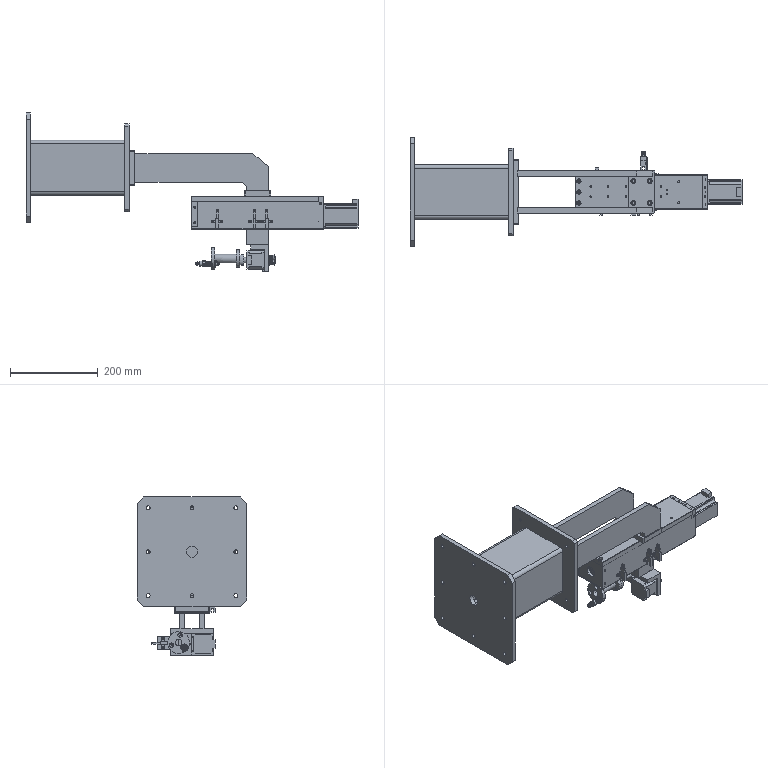Assembly | SolidWorks | mm | 44 component files | 44 solids | 4074 faces | box 757 x 250 x 360.5 mm | volume 3557328 mm3 | plane 1934 | cylinder 1155 | spline 581 | cone 270 | torus 110 | sphere 24 | commonest cylinder face diameters 0.56 x124 0.3 x118 3.95 x112 3.3 x54 19.94 x54 2 x50 4.2 x48 22.16 x48
Bill of materials:
6000Bearing | 2 |  | Thick flat ring (annular washer/spacer shape) with a central through-hole; outer diameter roughly 2.5x the bore, axial thickness roughly a third of the outer diameter.
628Bearing | 1 |  | Thick annular disc/spacer with a central through-hole that is smaller relative to the outer diameter than in a typical washer (bore about one third of OD).
angular contact ball bearings gb | 1 |  | Assembly shaped like a radial ball bearing: outer ring, inner ring with central bore, and a ring of about 13 spherical balls between them, with no cage or shields visible.
Base | 1 | Plain Carbon Steel | Spool-like bracket: a hollow-looking rectangular box/tube body joining two flat end plates of different sizes. The plates have chamfered corners, a pattern of small holes near the edges and one larger central hole on the end plate.
BNK1208-2-Nut | 1 |  | Flanged cylindrical bushing/nut-like body: a long cylindrical barrel with a thicker flange at one end. The flange is round with two flat-cut sides, has four through-holes, and there is a central through-bore.
BNK1208-2-ScrewRod | 1 |  | Long slender stepped round shaft: a long main diameter, a short larger-diameter collar near one end, then several smaller stepped journals out to that end, plus a short reduced step at the opposite end.
CylinderConnectionPlate | 1 |  | Flanged stepped shaft: an oval/rounded-rectangular flange with two flat sides and two diagonally opposed through-holes, from which a stepped cylindrical shaft extends. The shaft has a small groove between steps and a bore in its free end. A small cross-hole sits in the flange edge and a countersunk-looking central hole is on the flange face.
Gewindestift_DIN_913_M3x3 | 4 |  | Short solid cylinder (pin/slug shape) with chamfered edges on both ends; length slightly greater than diameter.
Handball42-40Stepping | 1 |  | Square-bodied motor-like housing: a square cross-section body with chamfered corners and recessed side bands. The front face has four corner holes, a raised circular pilot boss and a protruding cylindrical output shaft with a flat. A rectangular block sticks out from one side near the rear.
HTPA24S3M100_A_P5_a | 1 |  | Toothed pulley shape: a cylindrical body with many axial teeth around its circumference, flanges on both sides with angled outer edges, a central through-bore, and one radial hole through the toothed hub.
HTPA24S3M100_A_P5_a | 1 |  | Cylindrical toothed wheel with evenly spaced straight axial teeth around its outside, a flange at each end, and a round central bore. The shape looks like a flanged toothed (timing-style) pulley.
MCGS32-8Coupler-2 | 1 |  | Cylindrical spacer/standoff-like sleeve with a small central through-hole; length roughly equal to the outer diameter.
Motor-57 | 1 |  | Elongated square-section motor-like body: a front mounting flange with rounded corners and four corner through-holes, a short pilot step and a plain cylindrical output shaft. Longitudinal grooves run along the body edges, and a rectangular block protrudes from the top near the rear end.
MountingPlate | 1 |  | L-shaped angle bracket: a plain horizontal top flange and a thicker perforated vertical flange.
NETWS3 | 1 |  | Thin, flat, open ring with one wide radial gap and two inner notches. The outline looks like an E-style retaining clip.
NutFlatWasher | 1 |  | Rectangular block with one round through-hole in the middle of its largest face.
NutRubberPad | 1 |  | Thick cylindrical ring or spacer with a centred through-bore.
Part7RobotArmBase-Copy | 1 |  | Flat rectangular plate with chamfered corners, a long obround slot pair at each end, and two columns of three round holes.
RobotArmCrossPlate1 | 2 |  | Flat bar with a straight main section and one shaped end: an angled edge plus a small stepped notch.
RobotArmSupportPlate | 1 |  | Rectangular plate with small corner chamfers and four round holes in a rectangular pattern.
SensorPlate7 | 1 |  | Sheet-metal style L-bracket with an inside bend radius and rounded outer corners.
ServoVerticalBasePlate-2 | 1 |  | Long rectangular plate with two shallow transverse grooves across the top and many holes of several sizes.
SRK1010_nut_nut | 2 |  | Thin hexagonal nut-like part with chamfered corners and a large round central bore.
SRK1010_nut_spring | 1 |  | Open-coiled helical coil of round wire, roughly four to five turns, with a constant coil diameter.
SRK1010 | 1 |  | Stepped axial shaft carrying a square or hex block with a cross-hole and a separate hex nut. Both ends have short reduced-diameter stubs with grooves.
SRS15WM-240GuideRail-2 | 1 |  | Long, thin rectangular bar or plate with two parallel rows of five evenly spaced round through holes, and a lengthwise groove with angled walls along each long side.
SRS15WM-Slider-2 | 1 |  | Rectangular block with a wide, shallow, flat-bottomed channel cut across its full length, leaving a raised lip along each edge (a U-shaped profile). The edges are lightly chamfered.
SuctionCupBracket | 1 |  | Spool-shaped turned part: a cylindrical tube with a circular flange at each end, the two flanges of different diameters. A central through bore runs along the axis, and each flange has a ring of three holes.
UpperServoSeat-2 | 1 |  | Thick rectangular plate with a large round through bore in its lower centre. Three round holes run in a row along the top of the front face. The top edge has two small holes, one side face has a small hole, one side has a step, and the two bottom corners are chamfered.
U-shapedSensor | 3 |  | Upright body with an open U-shaped slot (fork) at its lower end and a stepped narrower upper section. Three thin parallel flat tabs, each with a hole near its tip, project from the top. A side arm or flange carries two oblong slotted holes.
U-shapedSensor8.28 | 1 |  | Body similar to the previous fork-shaped part: an open U-slot at one end, a stepped middle section, and three thin flat tabs with holes at the tips. A perpendicular flange carries two oblong slotted holes. The flange arrangement seen in these views differs from the previous part.
VerticalFrontSeat-2 | 1 |  | T-shaped block: a wide rectangular top flange with two vertical through holes sits on a narrower body. The body has a large horizontal round through bore with an internal step or groove, and its two lower corners are chamfered.
VerticalNutSeat-2 | 1 |  | Rectangular block with a large round bore through its front face, surrounded by four small blind holes in a square pattern. The top face has four through holes and a raised lip along each edge. The lower part is split by a wide open slot into two legs.
VerticalRearSeat-2 | 1 |  | Thick rectangular plate with a central round through bore. The top edge has three small holes and one side edge has two small holes, and the two bottom corners are chamfered.
VerticalSideCoverPlate-2 | 1 |  | Thin-walled U-channel, likely sheet metal, with two tall side walls and a flat base. Each side wall has round holes near its ends and small holes along it. The base has two long parallel slots with rounded ends and one round hole.
VPDT6 | 1 |  | Solid of revolution with stepped and contoured outside. A large plain cylinder with a central bore leads into a cone that narrows to a small rounded neck groove. Next comes a rounded ridge, then a second cone that narrows to a thin small-diameter disc or collar at the far end.
Mates:
1. coincident | ServoVerticalBasePlate-2-1 face at (94.478, -18.055, 48.551) dir (1, 0, 0) | UpperServoSeat-2-1 face at (94.478, -18.055, 48.551) dir (-1, 0, 0)
2. coincident | ServoVerticalBasePlate-2-1 face at (-195.522, -18.055, 36.551) dir (0, 0, -1) | UpperServoSeat-2-1 face at (94.478, -18.055, 36.551) dir (0, 0, 1)
3. coincident | ServoVerticalBasePlate-2-1 face at (-195.522, 57.945, 48.551) dir (0, 1, 0) | UpperServoSeat-2-1 face at (92.478, 57.945, 48.551) dir (0, 1, 0)
4. coincident | ServoVerticalBasePlate-2-1 face at (-195.522, -18.055, 36.551) dir (0, 0, -1) | VerticalRearSeat-2-1 face at (-181.522, 57.945, 36.551) dir (0, 0, 1)
5. coincident | ServoVerticalBasePlate-2-1 face at (-195.522, 57.945, 48.551) dir (0, 1, 0) | VerticalRearSeat-2-1 face at (-181.522, 57.945, 36.551) dir (0, 1, 0)
6. coincident | ServoVerticalBasePlate-2-1 face at (-195.522, -18.055, 48.551) dir (-1, 0, 0) | VerticalRearSeat-2-1 face at (-195.522, 57.945, 36.551) dir (-1, 0, 0)
7. concentric | ServoVerticalBasePlate-2-1 face at (39.478, 43.945, 36.551) dir (0, 0, -1) r 2.5 | VerticalFrontSeat-2-1 face at (39.478, 43.945, 38.551) dir (0, 0, -1) r 3.5
8. concentric | ServoVerticalBasePlate-2-1 face at (39.478, -4.055, 36.551) dir (0, 0, -1) r 2.5 | VerticalFrontSeat-2-1 face at (39.478, -4.055, 38.551) dir (0, 0, -1) r 3.5
9. coincident | ServoVerticalBasePlate-2-1 face at (-195.522, -18.055, 36.551) dir (0, 0, -1) | VerticalFrontSeat-2-1 face at (28.978, -10.055, 36.551) dir (0, 0, 1)
10. concentric | VerticalFrontSeat-2-1 face at (36.978, 19.945, 3.551) dir (-1, 0, 0) r 13 | 6000Bearing-1 face at (36.978, 19.945, 3.551) dir (-1, 0, 0) r 13
11. coincident | VerticalFrontSeat-2-1 face at (28.978, -10.055, 36.551) dir (-1, 0, 0) | 6000Bearing-1 face at (28.978, 19.945, 3.551) dir (-1, 0, 0)
12. concentric | VerticalFrontSeat-2-1 face at (41.978, 19.945, 3.551) dir (1, 0, 0) r 13 | 6000Bearing-2 face at (41.978, 19.945, 3.551) dir (1, 0, 0) r 13
13. coincident | VerticalFrontSeat-2-1 face at (49.978, -10.055, 36.551) dir (1, 0, 0) | 6000Bearing-2 face at (49.978, 19.945, 3.551) dir (1, 0, 0)
14. concentric | 6000Bearing-1 face at (36.978, 19.945, 3.551) dir (-1, 0, 0) r 5 | BNK1208-2-ScrewRod-1 face at (28.978, 19.945, 3.551) dir (1, 0, 0) r 5
15. coincident | 6000Bearing-1 face at (28.978, 19.945, 3.551) dir (-1, 0, 0) | BNK1208-2-ScrewRod-1 face at (28.978, 19.945, 3.551) dir (1, 0, 0)
16. coincident | ServoVerticalBasePlate-2-1 face at (-195.522, -18.055, 36.551) dir (0, 0, -1) | SRS15WM-240GuideRail-2-2 face at (18.478, 40.945, 36.551) dir (0, 0, 1)
17. coincident | SRS15WM-240GuideRail-2-2 face at (18.478, 40.945, 27.051) dir (0, 0, -1) | SRS15WM-Slider-2-1 face at (-73.445, -1.055, 27.051) dir (0, 0, 1)
18. coincident | SRS15WM-240GuideRail-2-2 face at (18.478, -1.055, 36.551) dir (0, -1, 0) | SRS15WM-Slider-2-1 face at (-73.445, -1.055, 33.151) dir (0, 1, 0)
19. concentric | BNK1208-2-ScrewRod-1 face at (-181.022, 19.945, 3.551) dir (1, 0, 0) r 6 | BNK1208-2-Nut-1 face at (-56.695, 19.945, 3.551) dir (1, 0, 0) r 14.5
20. parallel | SRS15WM-Slider-2-1 face at (-73.445, -10.055, 20.551) dir (0, 0, -1) | BNK1208-2-Nut-1 face at (-60.695, 35.765, -12.449) dir (0, 0, -1)
21. coincident | SRS15WM-Slider-2-1 face at (-73.445, -10.055, 20.551) dir (0, 0, -1) | VerticalNutSeat-2-1 face at (-20.695, 49.945, 20.551) dir (0, 0, 1)
22. coincident | SRS15WM-Slider-2-1 face at (-73.445, 49.945, 33.151) dir (0, 1, 0) | VerticalNutSeat-2-1 face at (-70.695, 49.945, 24.551) dir (0, -1, 0)
23. concentric | SRS15WM-Slider-2-1 face at (-35.695, -2.555, 20.551) dir (0, 0, -1) r 1.65 | VerticalNutSeat-2-1 face at (-35.695, -2.555, -27.449) dir (0, 0, -1) r 2.25
24. coincident | BNK1208-2-Nut-1 face at (-20.695, 19.945, 3.551) dir (-1, 0, 0) | VerticalNutSeat-2-1 face at (-20.695, 49.945, -27.449) dir (1, 0, 0)
25. concentric | BNK1208-2-ScrewRod-1 face at (58.978, 19.945, 3.551) dir (1, 0, 0) r 4 | MCGS32-8Coupler-2-1 face at (92.978, 19.945, 3.551) dir (-1, 0, 0) r 16
26. distance | MCGS32-8Coupler-2-1 face at (63.978, 19.945, 3.551) dir (-1, 0, 0) | BNK1208-2-ScrewRod-1 face at (73.978, 19.945, 3.551) dir (1, 0, 0)
27. coincident | UpperServoSeat-2-1 face at (92.478, -18.055, 48.551) dir (0, -1, 0) | VerticalSideCoverPlate-2-1 face at (-195.522, -18.055, 47.551) dir (0, 1, 0)
28. coincident | UpperServoSeat-2-1 face at (92.478, -18.055, -26.449) dir (0, 0, -1) | VerticalSideCoverPlate-2-1 face at (-195.522, -19.055, -26.449) dir (0, 0, 1)
29. coincident | UpperServoSeat-2-1 face at (104.478, -18.055, 48.551) dir (1, 0, 0) | VerticalSideCoverPlate-2-1 face at (104.478, -17.955, -26.449) dir (1, 0, 0)
30. coincident | VerticalRearSeat-2-1 face at (-181.522, 57.945, 36.551) dir (1, 0, 0) | SRS15WM-240GuideRail-2-2 face at (-181.522, 40.945, 36.551) dir (-1, 0, 0)
31. concentric | VerticalSideCoverPlate-2-1 face at (-148.022, -19.055, -9.449) dir (0, -1, 0) r 1.25 | U-shapedSensor-1 face at (-148.022, -32.655, -9.449) dir (0, 1, 0) r 1.6
32. concentric | VerticalSideCoverPlate-2-1 face at (-128.522, -19.055, -9.449) dir (0, -1, 0) r 1.25 | U-shapedSensor-1 face at (-128.522, -32.655, -9.449) dir (0, 1, 0) r 1.6
33. coincident | VerticalSideCoverPlate-2-1 face at (-195.522, -19.055, 47.551) dir (0, -1, 0) | U-shapedSensor-1 face at (-134.472, -19.055, -25.349) dir (0, 1, 0)
34. concentric | VerticalSideCoverPlate-2-1 face at (-63.022, -19.055, -9.449) dir (0, -1, 0) r 1.25 | U-shapedSensor-2 face at (-63.022, -32.655, -9.449) dir (0, 1, 0) r 1.6
35. concentric | VerticalSideCoverPlate-2-1 face at (-43.522, -19.055, -9.449) dir (0, -1, 0) r 1.25 | U-shapedSensor-2 face at (-43.522, -32.655, -9.449) dir (0, 1, 0) r 1.6
36. coincident | VerticalSideCoverPlate-2-1 face at (-195.522, -19.055, 47.551) dir (0, -1, 0) | U-shapedSensor-2 face at (-49.472, -19.055, -25.349) dir (0, 1, 0)
37. concentric | VerticalSideCoverPlate-2-1 face at (-35.022, -19.055, -9.449) dir (0, -1, 0) r 1.25 | U-shapedSensor-3 face at (-35.022, -32.655, -9.449) dir (0, 1, 0) r 1.6
38. concentric | VerticalSideCoverPlate-2-1 face at (-15.522, -19.055, -9.449) dir (0, -1, 0) r 1.25 | U-shapedSensor-3 face at (-15.522, -32.655, -9.449) dir (0, 1, 0) r 1.6
39. coincident | VerticalSideCoverPlate-2-1 face at (-195.522, -19.055, 47.551) dir (0, -1, 0) | U-shapedSensor-3 face at (-21.472, -19.055, -25.349) dir (0, 1, 0)
40. coincident | UpperServoSeat-2-1 face at (104.478, -18.055, 48.551) dir (1, 0, 0) | Motor-57-1 face at (104.478, 48.145, -24.649) dir (-1, 0, 0)
41. concentric | Motor-57-1 face at (83.878, 19.945, 3.551) dir (1, 0, 0) r 4 | UpperServoSeat-2-1 face at (89.478, 19.945, 3.551) dir (1, 0, 0) r 19.1
42. parallel | UpperServoSeat-2-1 face at (92.478, -18.055, -26.449) dir (0, 0, -1) | Motor-57-1 face at (104.478, 48.145, -24.649) dir (0, 0, -1)
43. concentric | BNK1208-2-ScrewRod-1 face at (-191.022, 19.945, 3.551) dir (1, 0, 0) r 4 | 628Bearing-1 face at (-181.022, 19.945, 3.551) dir (-1, 0, 0) r 12
44. coincident | BNK1208-2-ScrewRod-1 face at (-181.022, 19.945, 3.551) dir (-1, 0, 0) | 628Bearing-1 face at (-181.022, 19.945, 3.551) dir (1, 0, 0)
45. concentric | BNK1208-2-ScrewRod-1 face at (-181.022, 19.945, 3.551) dir (1, 0, 0) r 6 | VerticalNutSeat-2-1 face at (-20.695, 19.945, 3.551) dir (-1, 0, 0) r 14.5
46. concentric | BNK1208-2-ScrewRod-1 face at (-181.022, 19.945, 3.551) dir (1, 0, 0) r 6 | NutRubberPad-1 face at (28.978, 19.945, 3.551) dir (-1, 0, 0) r 20
47. coincident | VerticalFrontSeat-2-1 face at (28.978, -10.055, 36.551) dir (-1, 0, 0) | NutRubberPad-1 face at (28.978, 19.945, 3.551) dir (1, 0, 0)
48. concentric | BNK1208-2-ScrewRod-1 face at (-181.022, 19.945, 3.551) dir (1, 0, 0) r 6 | NutFlatWasher-1 face at (-166.522, 19.945, 3.551) dir (-1, 0, 0) r 6
49. coincident | VerticalRearSeat-2-1 face at (-181.522, 57.945, 36.551) dir (1, 0, 0) | NutFlatWasher-1 face at (-181.522, -1.055, 24.551) dir (-1, 0, 0)
50. parallel | VerticalRearSeat-2-1 face at (-181.522, 57.945, -23.449) dir (0, 0, -1) | NutFlatWasher-1 face at (-166.522, -1.055, -17.449) dir (0, 0, -1)
51. coincident | ServoVerticalBasePlate-2-1 face at (-195.522, -18.055, 48.551) dir (0, 0, 1) | RobotArmSupportPlate-1 face at (-45.522, 19.945, 48.551) dir (0, 0, -1)
52. width | RobotArmSupportPlate-1 face at (-15.522, 69.945, 60.551) dir (0, 1, 0) | RobotArmSupportPlate-1 face at (-15.522, -30.055, 60.551) dir (0, -1, 0) | VerticalSideCoverPlate-2-1 face at (-195.522, 58.945, -27.449) dir (0, 1, 0) | VerticalSideCoverPlate-2-1 face at (-195.522, -19.055, 47.551) dir (0, -1, 0)
53. distance | RobotArmSupportPlate-1 face at (-15.522, 69.945, 60.551) dir (1, 0, 0) | UpperServoSeat-2-1 face at (104.478, -18.055, 48.551) dir (1, 0, 0)
54. distance | RobotArmSupportPlate-1 face at (-15.522, 69.945, 60.551) dir (0, 1, 0) | RobotArmCrossPlate1-1 face at (-174.022, 67.945, 113.051) dir (0, 1, 0)
55. coincident | RobotArmSupportPlate-1 face at (-45.522, 19.945, 60.551) dir (0, 0, 1) | RobotArmCrossPlate1-1 face at (-20.522, 67.945, 60.551) dir (0, 0, -1)
56. distance | RobotArmCrossPlate1-1 face at (-20.522, 55.945, 145.551) dir (1, 0, 0) | RobotArmSupportPlate-1 face at (-15.522, 69.945, 60.551) dir (1, 0, 0)
57. coincident | RobotArmCrossPlate1-1 face at (-20.522, 55.945, 145.551) dir (1, 0, 0) | RobotArmCrossPlate1-2 face at (-20.522, -28.055, 145.551) dir (1, 0, 0)
58. coincident | RobotArmSupportPlate-1 face at (-45.522, 19.945, 60.551) dir (0, 0, 1) | RobotArmCrossPlate1-2 face at (-20.522, -16.055, 60.551) dir (0, 0, -1)
59. width | Part7RobotArmBase-Copy-1 face at (-326.522, -55.055, 153.051) dir (0, -1, 0) | Part7RobotArmBase-Copy-1 face at (-326.522, 94.945, 153.051) dir (0, 1, 0) | RobotArmCrossPlate1-1 face at (-174.022, 67.945, 113.051) dir (0, 1, 0) | RobotArmCrossPlate1-2 face at (-174.022, -28.055, 113.051) dir (0, -1, 0)
60. distance | RobotArmCrossPlate1-2 face at (-174.022, -16.055, 113.051) dir (0, 1, 0) | RobotArmCrossPlate1-1 face at (-174.022, 67.945, 113.051) dir (0, 1, 0)
61. coincident | RobotArmCrossPlate1-1 face at (-327.522, 55.945, 145.551) dir (-1, 0, 0) | Part7RobotArmBase-Copy-1 face at (-327.522, 19.945, 113.051) dir (1, 0, 0)
62. width | RobotArmCrossPlate1-1 face at (-20.522, 55.945, 145.551) dir (0, 0, 1) | RobotArmCrossPlate1-1 face at (-20.522, 55.945, 80.551) dir (0, 0, -1) | Part7RobotArmBase-Copy-1 face at (-326.522, -55.055, 73.051) dir (0, 0, -1) | Part7RobotArmBase-Copy-1 face at (-326.522, -55.055, 153.051) dir (0, 0, 1)
63. coincident | Part7RobotArmBase-Copy-1 face at (-338.522, 19.945, 113.051) dir (-1, 0, 0) | Base-1 face at (-338.522, 19.945, 113.051) dir (1, 0, 0)
64. distance | Part7RobotArmBase-Copy-1 face at (-326.522, -55.055, 153.051) dir (0, -1, 0) | Base-1 face at (-338.522, -80.055, 213.051) dir (0, -1, 0)
65. distance | Part7RobotArmBase-Copy-1 face at (-326.522, -55.055, 153.051) dir (0, 0, 1) | Base-1 face at (-338.522, 119.945, 213.051) dir (0, 0, 1)
66. concentric | MountingPlate-1 face at (-32.695, 50.945, -97.449) dir (1, 0, 0) r 13 | angular contact ball bearings gb-1 face at (-27.702, 50.945, -97.449) dir (1, 0, 0) r 5.5
67. concentric | MountingPlate-1 face at (-20.695, -20.855, -112.949) dir (1, 0, 0) r 1.7 | Handball42-40Stepping-1 face at (-29.695, -20.855, -112.949) dir (1, 0, 0) r 1.25
68. coincident | MountingPlate-1 face at (-32.695, 50.945, -97.449) dir (1, 0, 0) | angular contact ball bearings gb-1 face at (-32.695, 48.888, -102.55) dir (-1, 0, 0)
69. parallel | MountingPlate-1 face at (-20.695, -29.055, -122.449) dir (0, -1, 0) | Handball42-40Stepping-1 face at (-69.695, -26.355, -118.449) dir (0, -1, 0)
70. concentric | angular contact ball bearings gb-1 face at (-27.702, 50.945, -97.449) dir (1, 0, 0) r 2 | CylinderConnectionPlate-1 face at (-24.695, 50.945, -97.449) dir (-1, 0, 0) r 4.5
71. coincident | angular contact ball bearings gb-1 face at (-28.695, 50.197, -99.304) dir (1, 0, 0) | CylinderConnectionPlate-1 face at (-28.695, 55.443, -97.589) dir (1, 0, 0)
72. coincident | VerticalNutSeat-2-1 face at (-20.695, 49.945, -62.449) dir (0, 0, -1) | MountingPlate-1 face at (-34.695, 70.945, -62.449) dir (0, 0, 1)
73. width | MountingPlate-1 face at (-20.695, -29.055, -122.449) dir (0, -1, 0) | MountingPlate-1 face at (-34.695, 68.945, -72.449) dir (0, 1, 0) | VerticalNutSeat-2-1 face at (-70.695, 47.445, -22.449) dir (0, 1, 0) | VerticalNutSeat-2-1 face at (-70.695, -7.555, -22.449) dir (0, -1, 0)
74. coincident | VerticalNutSeat-2-1 face at (-20.695, 49.945, -27.449) dir (1, 0, 0) | MountingPlate-1 face at (-20.695, 70.945, -72.449) dir (1, 0, 0)
75. coincident | CylinderConnectionPlate-1 face at (-86.695, 50.945, -97.449) dir (-1, 0, 0) | SuctionCupBracket-1 face at (-86.695, 50.381, -94.093) dir (1, 0, 0)
76. concentric | CylinderConnectionPlate-1 face at (-86.695, 64.55, -99.016) dir (-1, 0, 0) r 2.1 | SuctionCupBracket-1 face at (-93.695, 64.55, -99.016) dir (1, 0, 0) r 2.75
77. concentric | CylinderConnectionPlate-1 face at (-86.695, 40.658, -105.515) dir (-1, 0, 0) r 2.1 | SuctionCupBracket-1 face at (-93.695, 40.658, -105.515) dir (1, 0, 0) r 2.75
78. concentric | Handball42-40Stepping-1 face at (-9.695, -5.355, -97.449) dir (-1, 0, 0) r 2.5 | HTPA24S3M100_A_P5_a-1 face at (2.305, -5.355, -97.449) dir (-1, 0, 0) r 2.5
79. distance | HTPA24S3M100_A_P5_a-1 face at (-5.695, -2.026, -98.53) dir (1, 0, 0) | Handball42-40Stepping-1 face at (-9.695, -5.355, -97.449) dir (1, 0, 0)
80. concentric | CylinderConnectionPlate-1 face at (-6.695, 50.945, -97.449) dir (-1, 0, 0) r 4 | HTPA24S3M100_A_P5_a-2 face at (2.305, 50.945, -97.449) dir (-1, 0, 0) r 4
81. coincident | HTPA24S3M100_A_P5_a-1 face at (-5.695, -2.026, -98.53) dir (1, 0, 0) | HTPA24S3M100_A_P5_a-2 face at (-5.695, 52.473, -100.599) dir (1, 0, 0)
82. coincident | SensorPlate7-1 face at (-34.295, 68.945, -80.449) dir (-1, 0, 0) | U-shapedSensor8.28-1 face at (-34.295, 69.645, -92.249) dir (1, 0, 0)
83. width | U-shapedSensor8.28-1 face at (-37.295, 82.445, -82.449) dir (0, 0, 1) | U-shapedSensor8.28-1 face at (-37.295, 82.445, -108.449) dir (0, 0, -1) | SensorPlate7-1 face at (-33.095, 68.945, -110.449) dir (0, 0, -1) | SensorPlate7-1 face at (-34.295, 68.945, -80.449) dir (0, 0, 1)
84. distance | SensorPlate7-1 face at (-33.095, 68.945, -90.462) dir (0, -1, 0) | U-shapedSensor8.28-1 face at (-37.295, 82.445, -95.449) dir (0, -1, 0)
85. distance | SensorPlate7-1 face at (-33.095, 68.945, -110.449) dir (0, 0, -1) | MountingPlate-1 face at (-20.695, -29.055, -122.449) dir (0, 0, -1)
86. distance | MountingPlate-1 face at (-20.695, 70.945, -72.449) dir (1, 0, 0) | SensorPlate7-1 face at (-22.295, 68.945, -110.449) dir (1, 0, 0)
87. coincident | MountingPlate-1 face at (-34.695, 68.945, -72.449) dir (0, 1, 0) | SensorPlate7-1 face at (-33.095, 68.945, -90.462) dir (0, -1, 0)
88. coincident | SRK1010-1 axis at (-197.952, 37.141, -105.536) dir (1, 0, 0) | SRK1010_nut_nut-1 axis at (-92.195, 37.141, -105.536) dir (-1, 0, 0)
89. coincident | SRK1010-1 axis at (-197.952, 37.141, -105.536) dir (1, 0, 0) | SRK1010_nut_nut-2 axis at (-100.195, 37.141, -105.536) dir (-1, 0, 0)
90. coincident | SRK1010-1 plane at (-135.602, 37.141, -105.536) dir (-1, 0, 0) | NETWS3-1 plane at (-135.602, 37.141, -105.536) dir (1, 0, 0)
91. coincident | SRK1010-1 axis at (-197.952, 37.141, -105.536) dir (1, 0, 0) | NETWS3-1 axis at (-54.702, 37.141, -105.536) dir (-1, 0, 0)
92. coincident | SRK1010-1 axis at (-197.952, 37.141, -105.536) dir (1, 0, 0) | SRK1010_nut_spring-1 axis at (-113.952, 37.141, -105.536) dir (-1, 0, 0)
93. angle | SRK1010_nut_spring-1 plane at (-163.952, 37.141, -105.536) dir (0, -0.8017, -0.5978) | SRK1010-1 plane at (-147.952, 37.141, -105.536) dir (0, 0.8017, 0.5978)
94. distance | SRK1010_nut_nut-2 face at (-148.695, 37.141, -105.536) dir (1, 0, 0) | SRK1010_nut_nut-1 face at (-143.695, 42.38, -100.894) dir (-1, 0, 0)
95. concentric | SRK1010-1 face at (-132.052, 37.141, -105.536) dir (-1, 0, 0) r 2.5 | VPDT6-1 face at (-186.952, 37.141, -105.536) dir (1, 0, 0) r 2.5
96. coincident | SRK1010-1 face at (-171.952, 39.145, -104.042) dir (-1, 0, 0) | VPDT6-1 face at (-171.952, 37.141, -105.536) dir (1, 0, 0)
97. concentric | SuctionCupBracket-1 face at (-143.695, 37.141, -105.536) dir (-1, 0, 0) r 5 | SRK1010-1 face at (-132.052, 37.141, -105.536) dir (-1, 0, 0) r 4.188
98. coincident | SuctionCupBracket-1 face at (-143.695, 50.381, -94.093) dir (1, 0, 0) | SRK1010_nut_nut-1 face at (-143.695, 42.38, -100.894) dir (-1, 0, 0)